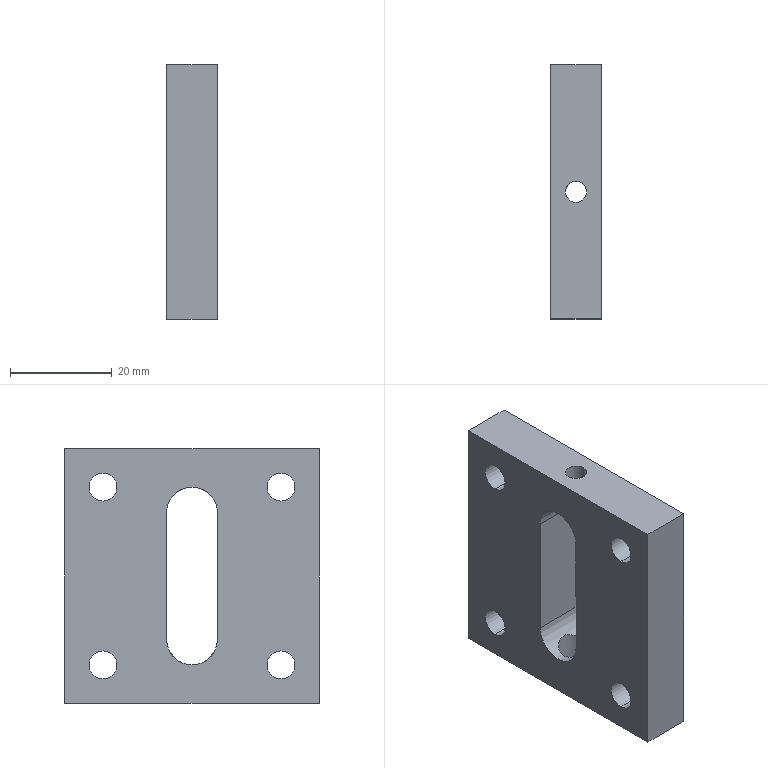Component | SolidWorks | 01-11CodingRubberRollerMountingPlate-1 | 1 solid | 35 faces | box 10 x 50 x 50 mm | volume 19121 mm3 | cylinder 23 | plane 12 | commonest cylinder face diameters 10 x11 5.5 x8 6.864 x2 4.2 x2 | material A3 Steel
build123d program:
from build123d import *

# Parameters (mm, degrees)
SKETCH1_W                                          = 50
SKETCH1_H                                          = 50
BOSS_EXTRUDE1_DEPTH                                = 5
CUT_EXTRUDE1_DEPTH                                 = 37.742
CUT_EXTRUDE1_DEPTH_BACK                            = 37.742
M5_TAPPED_HOLE1_D                                  = 4.2
HOLE_SIZE_ACCORDING_TO_TYPE_1_OF_HEXAG_D           = 5.5
HOLE_SIZE_ACCORDING_TO_TYPE_1_OF_HEXAG_CBORE_D     = 10
HOLE_SIZE_ACCORDING_TO_TYPE_1_OF_HEXAG_CBORE_DEPTH = 5.7
CUT_EXTRUDE2_REACH                                 = 58.125
CUT_EXTRUDE2_END_RADIUS                            = 5
SKETCH9_R                                          = 3.432


with BuildPart() as part:
    # Sketch1 → Boss-Extrude1 (new, symmetric)
    with BuildSketch(Plane.XY):
        Rectangle(SKETCH1_W, SKETCH1_H)
    extrude(amount=BOSS_EXTRUDE1_DEPTH, both=True)

    # Sketch2 → Cut-Extrude1 (cut, two sides: drawn at the far end of the back side and taken through both)
    with BuildSketch(Plane.XY.offset(5).offset(-CUT_EXTRUDE1_DEPTH_BACK)):
        with BuildLine():
            Line((-12.5, 5), (12.5, 5))
            ThreePointArc((12.5, 5), (17.5, 0), (12.5, -5))
            Line((12.5, -5), (-12.5, -5))
            ThreePointArc((-12.5, -5), (-17.5, 0), (-12.5, 5))
        make_face()
    extrude(amount=CUT_EXTRUDE1_DEPTH + CUT_EXTRUDE1_DEPTH_BACK, mode=Mode.SUBTRACT)

    # M5 Tapped Hole1 (through all)
    with Locations(Plane(origin=(25, 0, 0), x_dir=(0, 0, 1), z_dir=(1, 0, 0))):
        with Locations((0, 0)):
            Hole(M5_TAPPED_HOLE1_D / 2)

    # Hole Size _According to_ Type 1 of Hexag (through all)
    with Locations(Plane(origin=(-17.5, 17.5, 5), x_dir=(1, 0, 0), z_dir=(0, 0, 1))):
        with Locations((0, 0), (35, 0), (35, -35), (0, -35)):
            CounterBoreHole(HOLE_SIZE_ACCORDING_TO_TYPE_1_OF_HEXAG_D / 2, HOLE_SIZE_ACCORDING_TO_TYPE_1_OF_HEXAG_CBORE_D / 2, HOLE_SIZE_ACCORDING_TO_TYPE_1_OF_HEXAG_CBORE_DEPTH)

    # Cut-Extrude2: up to this cylinder (the profile starts outside it)
    cut_extrude2_end = Plane(origin=(-12.5, 0, 0), z_dir=(0, 0, 1)) * Cylinder(CUT_EXTRUDE2_END_RADIUS, 127.25, mode=Mode.PRIVATE)
    # Sketch9 → Cut-Extrude2 (cut, up to the surface)
    with BuildSketch(Plane.ZY.offset(25), mode=Mode.PRIVATE) as cut_extrude2_sk1:
        Circle(SKETCH9_R)
    cut_extrude2_tool1 = extrude(cut_extrude2_sk1.sketch, amount=-CUT_EXTRUDE2_REACH, mode=Mode.PRIVATE) - cut_extrude2_end
    add(cut_extrude2_tool1.solids().sort_by_distance((-25, 0, 0))[0], mode=Mode.SUBTRACT)


solid = part.part

# Placed as in the assembly
solid = solid.moved(Location((-441.91, 2.41, -2.5), (180, 90, 0)))